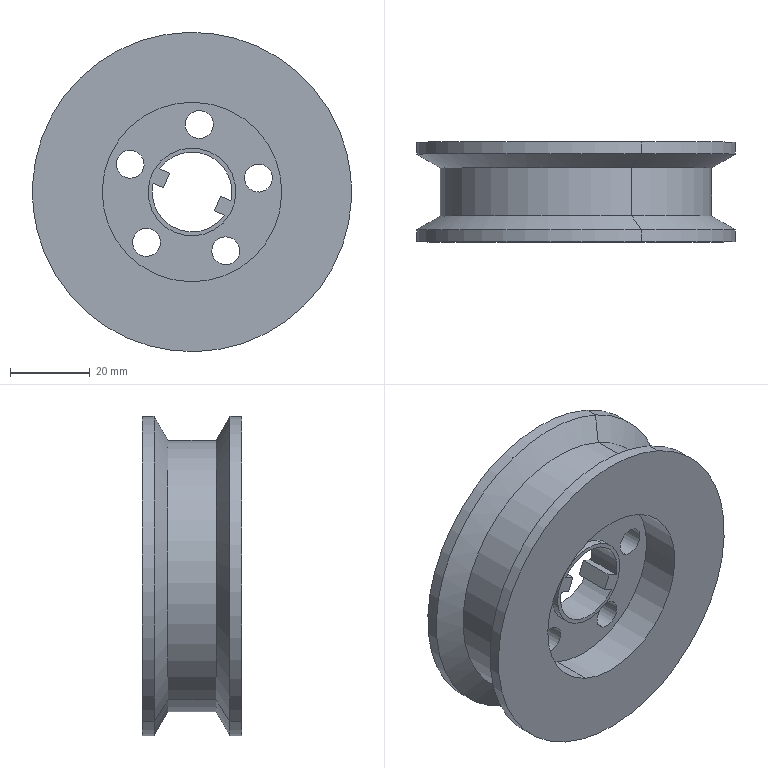Component | SolidWorks | LX-TSJ-08-1 | 1 solid | 43 faces | volume 69996 mm3 | cylinder 27 | plane 12 | cone 4 | commonest cylinder face diameters 7 x10 45 x4 80 x4 22 x4 20 x3 68 x2